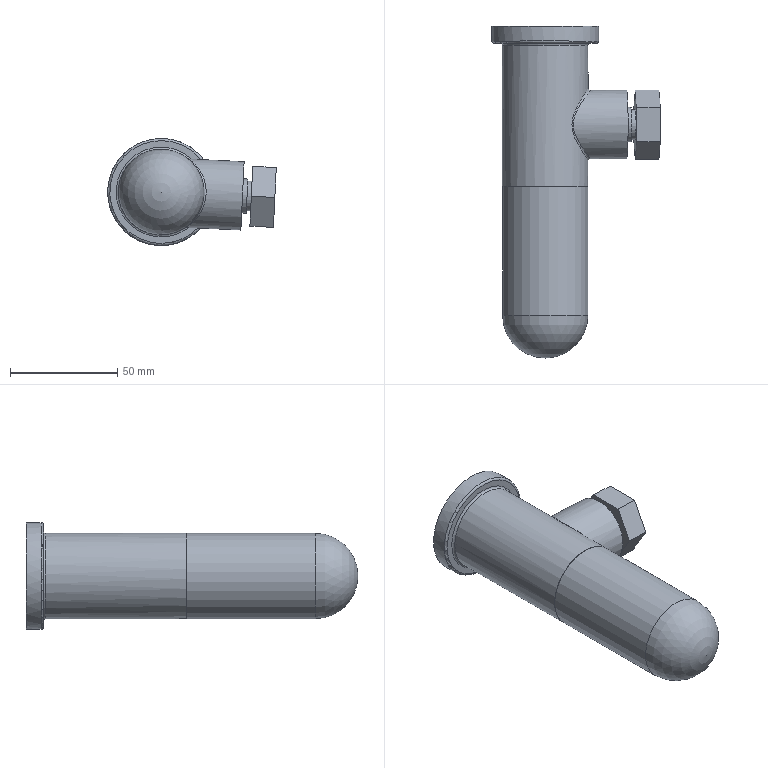Assembly | NX | mm | 6 component files | 6 solids | 66 faces | box 78.74 x 155 x 50 mm | volume 181533 mm3 | plane 30 | cylinder 15 | spline 9 | cone 6 | sphere 3 | torus 3 | commonest cylinder face diameters 22 x3 10 x3 40 x2 16 x2 50 x1 32 x1 30 x1 17 x1
Bill of materials:
unnamed part 1 | 1 |  | Short solid cylinder with a rounded, domed end and a flat end with a chamfer around it.
unnamed part 2 | 1 |  | Helical coil of round wire with a constant coil diameter and roughly eight evenly spaced open coils. The ends look closed and flattened.
unnamed part 3 | 1 |  | Stepped part with a hex head: a hexagonal prism head, a short narrow neck, a larger cylindrical step, and a smaller cylindrical end with a chamfer.
unnamed part 4 | 1 |  | Solid round rod with one rounded end (capsule-like) and a flat opposite end.
unnamed part 5 | 1 |  | Tee-shaped hollow fitting: a straight through-bore with a side branch at right angles, and a raised flange collar at one run end.
unnamed part 6 | 1 |  | Cylindrical pin with a conical pointed tip at one end and a small chamfer at the other. Near the chamfered end there is a tapered flat notch cut into one side.
Mates:
1. touch align | small_shaft 1 face | housing 1 face
2. touch align | liquid_column 1 face | small_shaft 1 face
3. touch align | liquid_column 1 face | small_shaft 1 face
4. touch align | locating_shaft 1 face | housing 1 face
5. touch align | spring 1 datumaxis | locating_shaft 1 face
6. touch align | liquid_column 1 face | locating_shaft 1 face
7. touch align | spring 1 datumplane | locating_shaft 1 face
8. touch align | top_shell 1 face | housing 1 face
9. touch align | top_shell 1 edge | housing 1 face